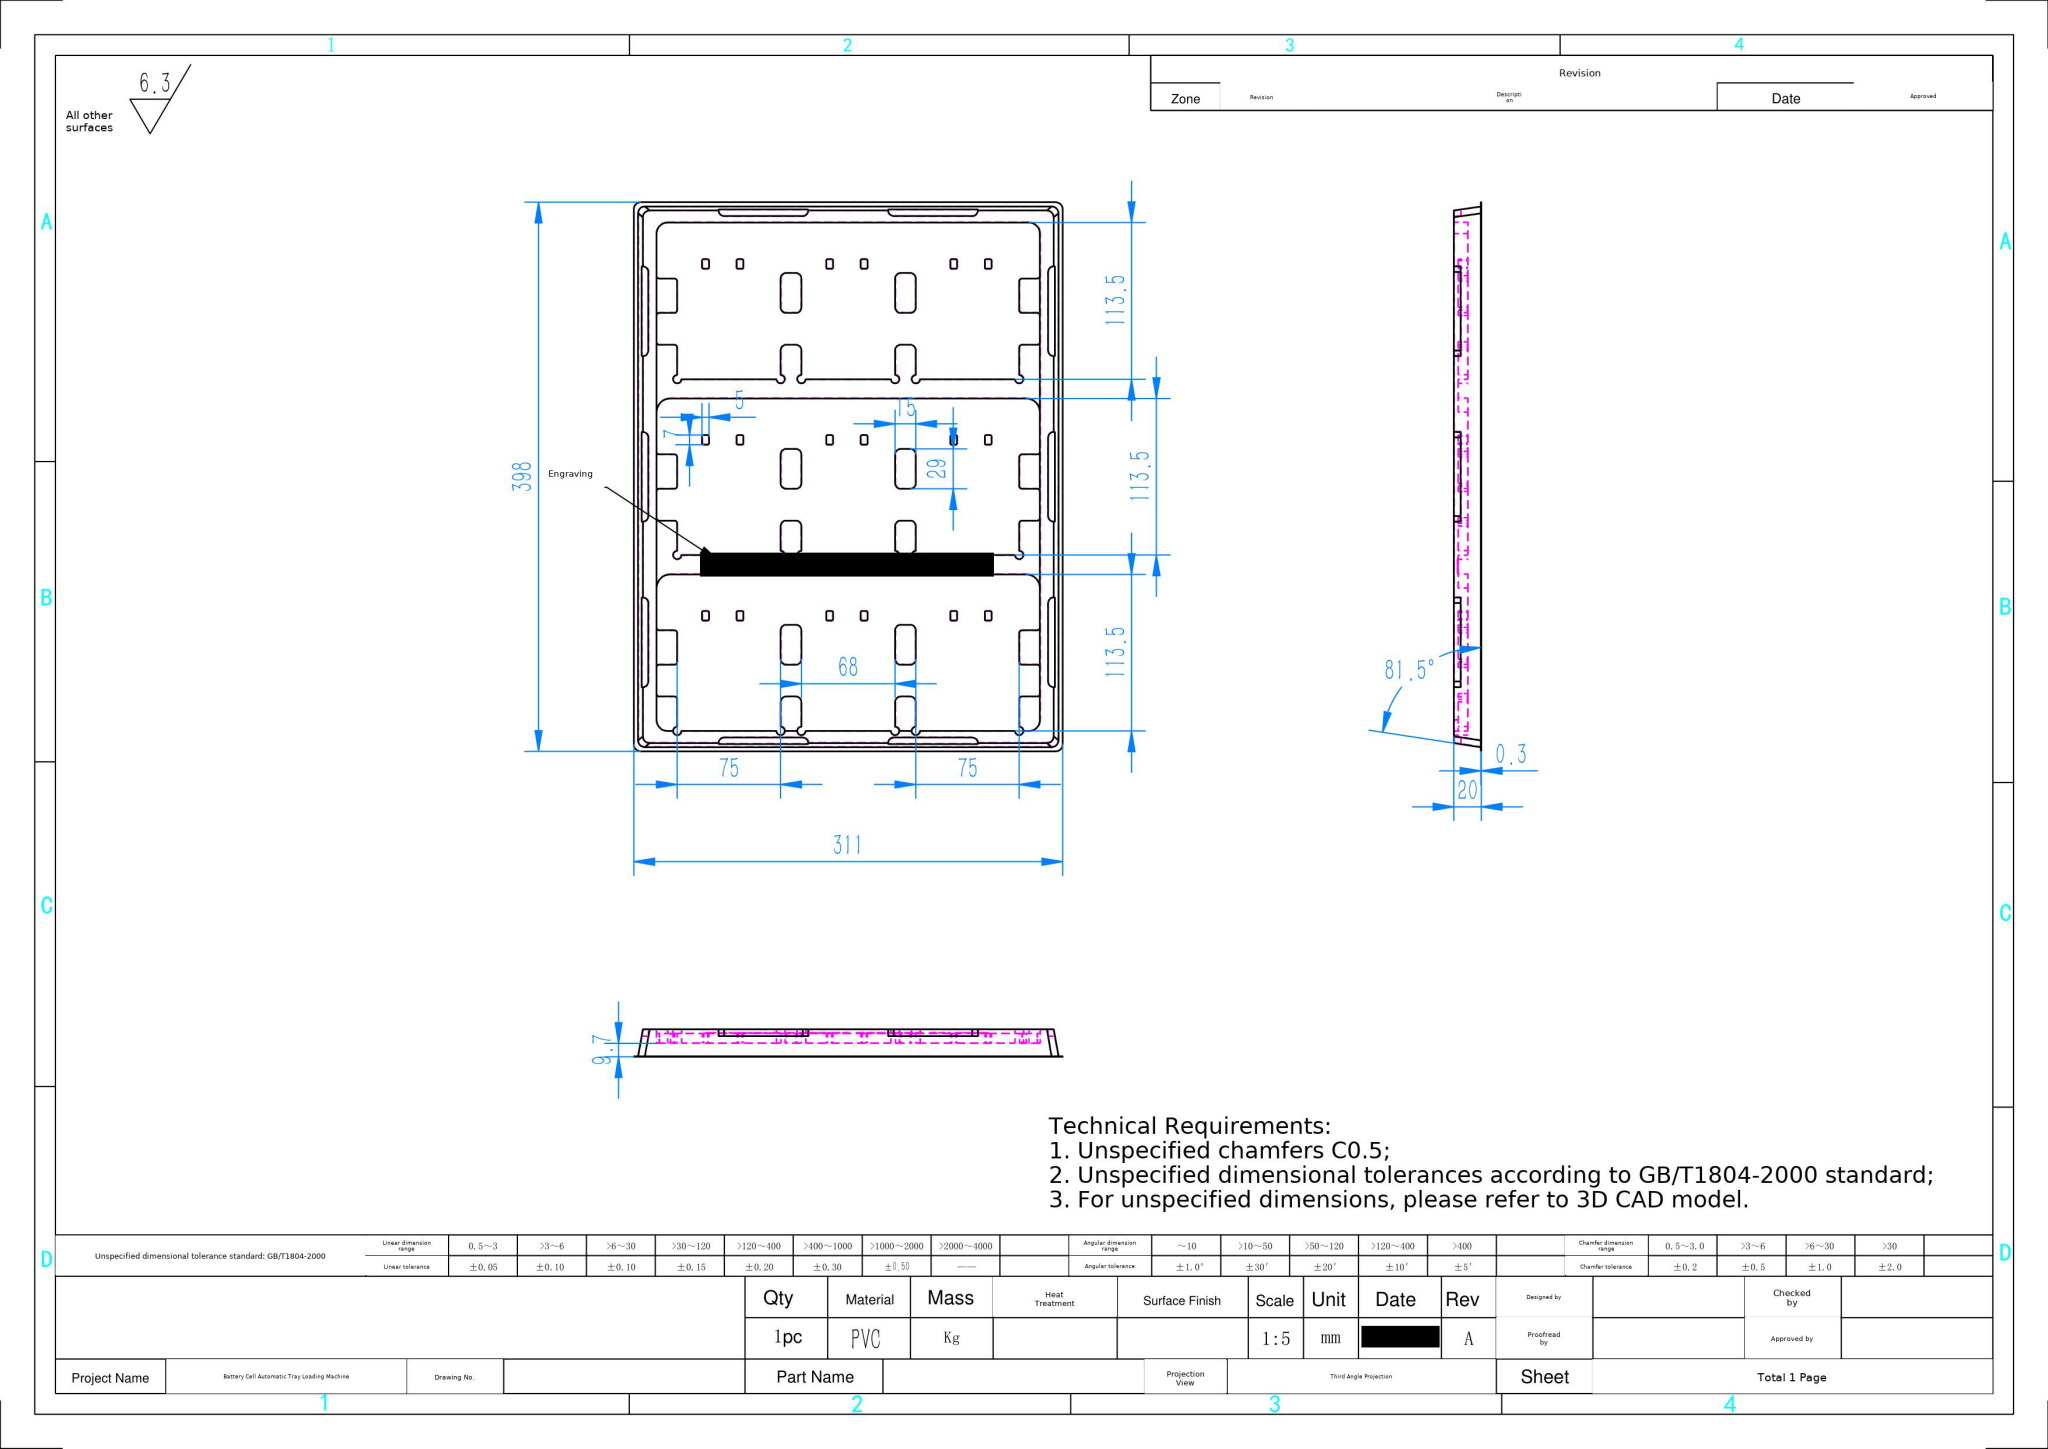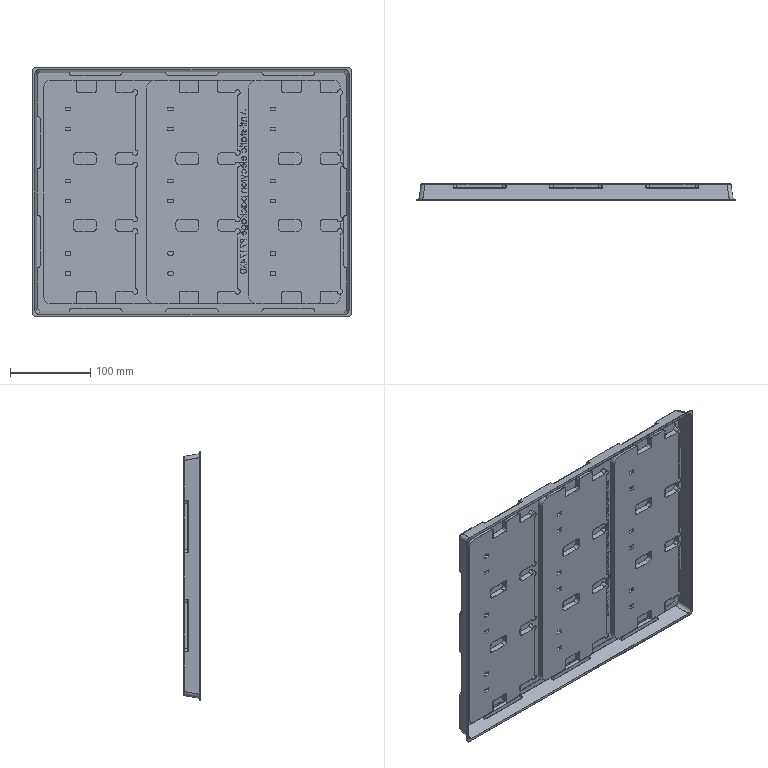Part | SolidWorks | mm | material PVC | 1 solid | 1711 faces | box 398 x 20 x 311 mm | volume 53463 mm3 | plane 944 | cylinder 418 | spline 349 | commonest cylinder face diameters 2 x72 1.4 x72 8 x60 4 x36 7.4 x36 6 x27 6.6 x27 8.6 x24